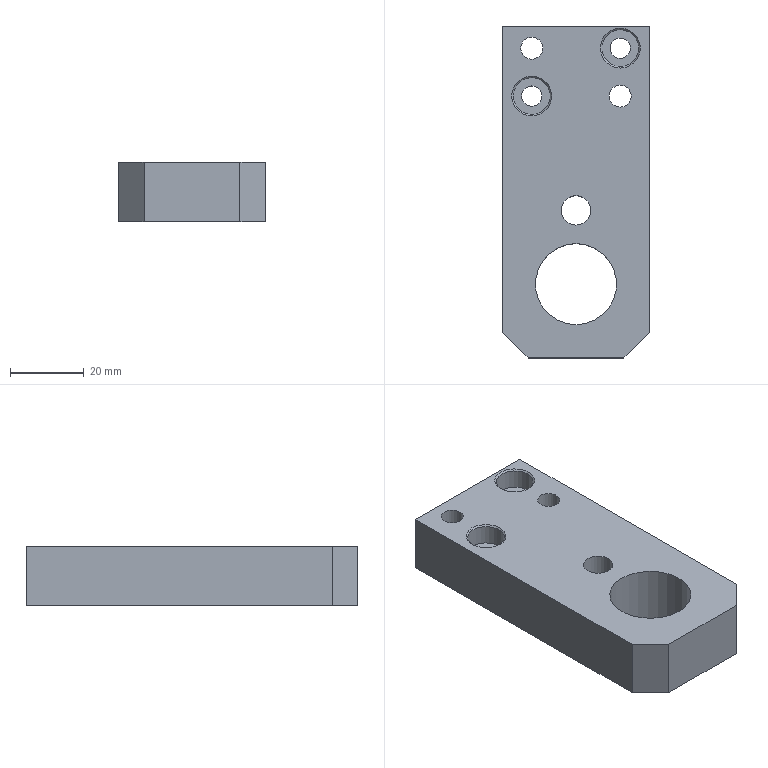Component | NX | DRILL_TEMPLATE | 1 solid | 22 faces | volume 47621 mm3 | plane 10 | cylinder 8 | cone 4 | commonest cylinder face diameters 5.5 x2 10 x2 6 x2 22 x1 8 x1